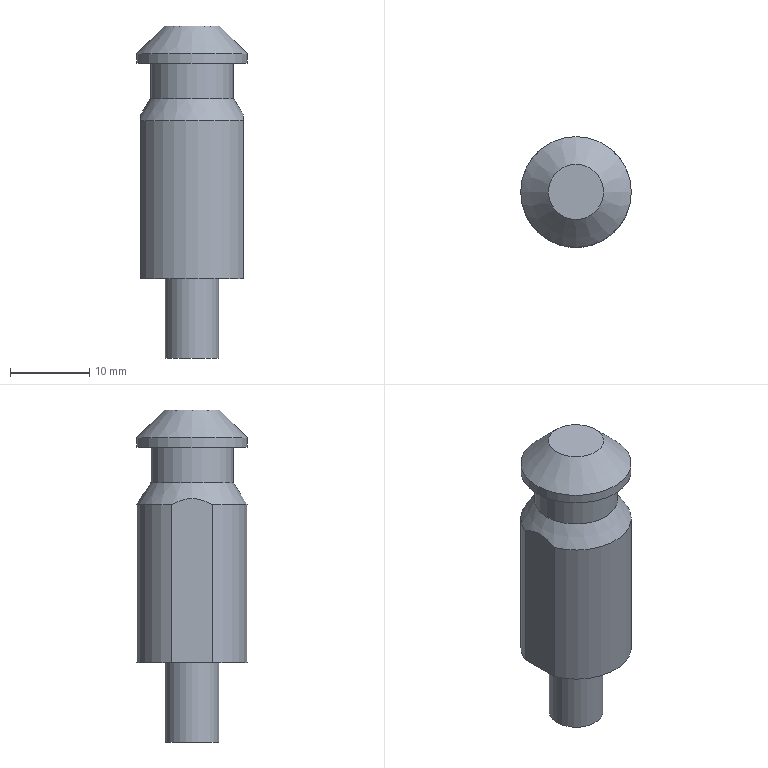Component | NX | PART | 1 solid | 13 faces | box 14 x 14 x 42 mm | volume 4592 mm3 | plane 6 | cylinder 5 | cone 2 | commonest cylinder face diameters 14 x3 6.8 x1 10.501 x1
STEP:
#1=CARTESIAN_POINT('',(0.,0.,0.));
#2=DIRECTION('',(0.,0.,1.));
#3=DIRECTION('',(1.,0.,0.));
#4=AXIS2_PLACEMENT_3D('',#1,#2,#3);
#5=CARTESIAN_POINT('',(-5.25,0.,31.8));
#6=VERTEX_POINT('',#5);
#7=CARTESIAN_POINT('',(-0.,0.,31.8));
#8=DIRECTION('',(0.,0.,-1.));
#9=DIRECTION('',(-1.,0.,0.));
#10=AXIS2_PLACEMENT_3D('',#7,#8,#9);
#11=CIRCLE('',#10,5.25);
#12=CARTESIAN_POINT('',(-0.,0.,31.8));
#13=DIRECTION('',(0.,0.,-1.));
#14=DIRECTION('',(-1.,0.,0.));
#15=AXIS2_PLACEMENT_3D('',#12,#13,#14);
#16=CONICAL_SURFACE('',#15,5.25,0.5585);
#17=CARTESIAN_POINT('',(0.,0.));
#18=DIRECTION('',(1.,0.));
#19=VECTOR('',#18,1.);
#20=LINE('',#17,#19);
#21=(GEOMETRIC_REPRESENTATION_CONTEXT(2)PARAMETRIC_REPRESENTATION_CONTEXT()REPRESENTATION_CONTEXT('',''));
#22=DEFINITIONAL_REPRESENTATION('',(#20),#21);
#23=PCURVE('',#16,#22);
#24=CARTESIAN_POINT('',(-0.,0.,9.));
#25=DIRECTION('',(0.,0.,-1.));
#26=DIRECTION('',(-1.,0.,0.));
#27=AXIS2_PLACEMENT_3D('',#24,#25,#26);
#28=CYLINDRICAL_SURFACE('',#27,5.25);
#29=CARTESIAN_POINT('',(0.,-22.8));
#30=DIRECTION('',(1.,0.));
#31=VECTOR('',#30,1.);
#32=LINE('',#29,#31);
#33=(GEOMETRIC_REPRESENTATION_CONTEXT(2)PARAMETRIC_REPRESENTATION_CONTEXT()REPRESENTATION_CONTEXT('',''));
#34=DEFINITIONAL_REPRESENTATION('',(#32),#33);
#35=PCURVE('',#28,#34);
#36=SURFACE_CURVE('',#11,(#23,#35),.PCURVE_S1.);
#37=EDGE_CURVE('',#6,#6,#36,.T.);
#38=ORIENTED_EDGE('',*,*,#37,.T.);
#39=CARTESIAN_POINT('',(-6.5,0.,29.8));
#40=VERTEX_POINT('',#39);
#41=CARTESIAN_POINT('',(-5.25,0.,31.8));
#42=CARTESIAN_POINT('',(-6.5,0.,29.8));
#43=B_SPLINE_CURVE_WITH_KNOTS('',1,(#41,#42),.UNSPECIFIED.,.F.,.F.,(2,2),(0.,2.358),.PIECEWISE_BEZIER_KNOTS.);
#44=CARTESIAN_POINT('',(6.283,0.));
#45=DIRECTION('',(0.,1.));
#46=VECTOR('',#45,1.);
#47=LINE('',#44,#46);
#48=(GEOMETRIC_REPRESENTATION_CONTEXT(2)PARAMETRIC_REPRESENTATION_CONTEXT()REPRESENTATION_CONTEXT('',''));
#49=DEFINITIONAL_REPRESENTATION('',(#47),#48);
#50=PCURVE('',#16,#49);
#51=CARTESIAN_POINT('',(0.,0.));
#52=DIRECTION('',(0.,1.));
#53=VECTOR('',#52,1.);
#54=LINE('',#51,#53);
#55=(GEOMETRIC_REPRESENTATION_CONTEXT(2)PARAMETRIC_REPRESENTATION_CONTEXT()REPRESENTATION_CONTEXT('',''));
#56=DEFINITIONAL_REPRESENTATION('',(#54),#55);
#57=PCURVE('',#16,#56);
#58=SEAM_CURVE('',#43,(#50,#57),.PCURVE_S1.);
#59=EDGE_CURVE('',#6,#40,#58,.T.);
#60=ORIENTED_EDGE('',*,*,#59,.T.);
#61=CARTESIAN_POINT('',(-6.5,-2.598,29.));
#62=VERTEX_POINT('',#61);
#63=CARTESIAN_POINT('',(-6.5,2.598,29.));
#64=CARTESIAN_POINT('',(-6.5,1.811,29.468));
#65=CARTESIAN_POINT('',(-6.5,0.9224,29.799));
#66=CARTESIAN_POINT('',(-6.5,-0.9091,29.802));
#67=CARTESIAN_POINT('',(-6.5,-1.805,29.471));
#68=CARTESIAN_POINT('',(-6.5,-2.598,29.));
#69=B_SPLINE_CURVE_WITH_KNOTS('',3,(#63,#64,#65,#66,#67,#68),.UNSPECIFIED.,.F.,.F.,(4,2,4),(0.,0.5,1.),.UNSPECIFIED.);
#70=CARTESIAN_POINT('',(6.663,2.8));
#71=CARTESIAN_POINT('',(6.654,2.757));
#72=CARTESIAN_POINT('',(6.635,2.675));
#73=CARTESIAN_POINT('',(6.604,2.558));
#74=CARTESIAN_POINT('',(6.572,2.45));
#75=CARTESIAN_POINT('',(6.54,2.351));
#76=CARTESIAN_POINT('',(6.506,2.262));
#77=CARTESIAN_POINT('',(6.471,2.185));
#78=CARTESIAN_POINT('',(6.435,2.12));
#79=CARTESIAN_POINT('',(6.398,2.068));
#80=CARTESIAN_POINT('',(6.361,2.029));
#81=CARTESIAN_POINT('',(6.323,2.006));
#82=CARTESIAN_POINT('',(6.284,1.997));
#83=CARTESIAN_POINT('',(6.246,2.005));
#84=CARTESIAN_POINT('',(6.208,2.028));
#85=CARTESIAN_POINT('',(6.17,2.066));
#86=CARTESIAN_POINT('',(6.133,2.118));
#87=CARTESIAN_POINT('',(6.097,2.183));
#88=CARTESIAN_POINT('',(6.062,2.26));
#89=CARTESIAN_POINT('',(6.028,2.349));
#90=CARTESIAN_POINT('',(5.995,2.448));
#91=CARTESIAN_POINT('',(5.963,2.556));
#92=CARTESIAN_POINT('',(5.932,2.674));
#93=CARTESIAN_POINT('',(5.912,2.757));
#94=CARTESIAN_POINT('',(5.903,2.8));
#95=B_SPLINE_CURVE_WITH_KNOTS('',3,(#70,#71,#72,#73,#74,#75,#76,#77,#78,#79,#80,#81,#82,#83,#84,#85,#86,#87,#88,#89,#90,#91,#92,#93,#94),.UNSPECIFIED.,.F.,.F.,(4,1,1,1,1,1,1,1,1,1,1,1,1,1,1,1,1,1,1,1,1,1,4),(0.,0.04545,0.09091,0.1364,0.1818,0.2273,0.2727,0.3182,0.3636,0.4091,0.4545,0.5,0.5455,0.5909,0.6364,0.6818,0.7273,0.7727,0.8182,0.8636,0.9091,0.9545,1.),.QUASI_UNIFORM_KNOTS.);
#96=(GEOMETRIC_REPRESENTATION_CONTEXT(2)PARAMETRIC_REPRESENTATION_CONTEXT()REPRESENTATION_CONTEXT('',''));
#97=DEFINITIONAL_REPRESENTATION('',(#95),#96);
#98=PCURVE('',#16,#97);
#99=CARTESIAN_POINT('',(-6.5,-6.7,35.5));
#100=DIRECTION('',(-1.,0.,0.));
#101=DIRECTION('',(0.,0.,1.));
#102=AXIS2_PLACEMENT_3D('',#99,#100,#101);
#103=PLANE('',#102);
#104=CARTESIAN_POINT('',(-6.5,9.298));
#105=CARTESIAN_POINT('',(-6.032,8.511));
#106=CARTESIAN_POINT('',(-5.701,7.622));
#107=CARTESIAN_POINT('',(-5.698,5.791));
#108=CARTESIAN_POINT('',(-6.029,4.895));
#109=CARTESIAN_POINT('',(-6.5,4.102));
#110=B_SPLINE_CURVE_WITH_KNOTS('',3,(#104,#105,#106,#107,#108,#109),.UNSPECIFIED.,.F.,.F.,(4,2,4),(0.,0.5,1.),.UNSPECIFIED.);
#111=(GEOMETRIC_REPRESENTATION_CONTEXT(2)PARAMETRIC_REPRESENTATION_CONTEXT()REPRESENTATION_CONTEXT('',''));
#112=DEFINITIONAL_REPRESENTATION('',(#110),#111);
#113=PCURVE('',#103,#112);
#114=SURFACE_CURVE('',#69,(#98,#113),.PCURVE_S1.);
#115=EDGE_CURVE('',#40,#62,#114,.T.);
#116=ORIENTED_EDGE('',*,*,#115,.T.);
#117=CARTESIAN_POINT('',(6.5,-2.598,29.));
#118=VERTEX_POINT('',#117);
#119=CARTESIAN_POINT('',(-0.,0.,29.));
#120=DIRECTION('',(0.,0.,-1.));
#121=DIRECTION('',(1.,0.,0.));
#122=AXIS2_PLACEMENT_3D('',#119,#120,#121);
#123=CIRCLE('',#122,7.);
#124=CARTESIAN_POINT('',(3.142,2.8));
#125=DIRECTION('',(1.,0.));
#126=VECTOR('',#125,1.);
#127=LINE('',#124,#126);
#128=(GEOMETRIC_REPRESENTATION_CONTEXT(2)PARAMETRIC_REPRESENTATION_CONTEXT()REPRESENTATION_CONTEXT('',''));
#129=DEFINITIONAL_REPRESENTATION('',(#127),#128);
#130=PCURVE('',#16,#129);
#131=CARTESIAN_POINT('',(-0.,0.,9.));
#132=DIRECTION('',(0.,0.,1.));
#133=DIRECTION('',(1.,0.,0.));
#134=AXIS2_PLACEMENT_3D('',#131,#132,#133);
#135=CYLINDRICAL_SURFACE('',#134,7.);
#136=CARTESIAN_POINT('',(6.283,20.));
#137=DIRECTION('',(-1.,0.));
#138=VECTOR('',#137,1.);
#139=LINE('',#136,#138);
#140=(GEOMETRIC_REPRESENTATION_CONTEXT(2)PARAMETRIC_REPRESENTATION_CONTEXT()REPRESENTATION_CONTEXT('',''));
#141=DEFINITIONAL_REPRESENTATION('',(#139),#140);
#142=PCURVE('',#135,#141);
#143=SURFACE_CURVE('',#123,(#130,#142),.PCURVE_S1.);
#144=EDGE_CURVE('',#118,#62,#143,.T.);
#145=ORIENTED_EDGE('',*,*,#144,.F.);
#146=CARTESIAN_POINT('',(6.5,2.598,29.));
#147=VERTEX_POINT('',#146);
#148=CARTESIAN_POINT('',(6.5,2.598,29.));
#149=CARTESIAN_POINT('',(6.5,1.811,29.468));
#150=CARTESIAN_POINT('',(6.5,0.9224,29.799));
#151=CARTESIAN_POINT('',(6.5,-0.9091,29.802));
#152=CARTESIAN_POINT('',(6.5,-1.805,29.471));
#153=CARTESIAN_POINT('',(6.5,-2.598,29.));
#154=B_SPLINE_CURVE_WITH_KNOTS('',3,(#148,#149,#150,#151,#152,#153),.UNSPECIFIED.,.F.,.F.,(4,2,4),(0.,0.5,1.),.UNSPECIFIED.);
#155=CARTESIAN_POINT('',(2.761,2.8));
#156=CARTESIAN_POINT('',(2.771,2.757));
#157=CARTESIAN_POINT('',(2.79,2.675));
#158=CARTESIAN_POINT('',(2.821,2.558));
#159=CARTESIAN_POINT('',(2.852,2.45));
#160=CARTESIAN_POINT('',(2.885,2.351));
#161=CARTESIAN_POINT('',(2.919,2.262));
#162=CARTESIAN_POINT('',(2.954,2.185));
#163=CARTESIAN_POINT('',(2.99,2.12));
#164=CARTESIAN_POINT('',(3.027,2.068));
#165=CARTESIAN_POINT('',(3.064,2.029));
#166=CARTESIAN_POINT('',(3.102,2.006));
#167=CARTESIAN_POINT('',(3.141,1.997));
#168=CARTESIAN_POINT('',(3.179,2.005));
#169=CARTESIAN_POINT('',(3.217,2.028));
#170=CARTESIAN_POINT('',(3.255,2.066));
#171=CARTESIAN_POINT('',(3.291,2.118));
#172=CARTESIAN_POINT('',(3.328,2.183));
#173=CARTESIAN_POINT('',(3.363,2.26));
#174=CARTESIAN_POINT('',(3.397,2.349));
#175=CARTESIAN_POINT('',(3.43,2.448));
#176=CARTESIAN_POINT('',(3.462,2.556));
#177=CARTESIAN_POINT('',(3.493,2.674));
#178=CARTESIAN_POINT('',(3.512,2.757));
#179=CARTESIAN_POINT('',(3.522,2.8));
#180=B_SPLINE_CURVE_WITH_KNOTS('',3,(#155,#156,#157,#158,#159,#160,#161,#162,#163,#164,#165,#166,#167,#168,#169,#170,#171,#172,#173,#174,#175,#176,#177,#178,#179),.UNSPECIFIED.,.F.,.F.,(4,1,1,1,1,1,1,1,1,1,1,1,1,1,1,1,1,1,1,1,1,1,4),(0.,0.04545,0.09091,0.1364,0.1818,0.2273,0.2727,0.3182,0.3636,0.4091,0.4545,0.5,0.5455,0.5909,0.6364,0.6818,0.7273,0.7727,0.8182,0.8636,0.9091,0.9545,1.),.QUASI_UNIFORM_KNOTS.);
#181=(GEOMETRIC_REPRESENTATION_CONTEXT(2)PARAMETRIC_REPRESENTATION_CONTEXT()REPRESENTATION_CONTEXT('',''));
#182=DEFINITIONAL_REPRESENTATION('',(#180),#181);
#183=PCURVE('',#16,#182);
#184=CARTESIAN_POINT('',(6.5,-6.7,35.5));
#185=DIRECTION('',(-1.,0.,0.));
#186=DIRECTION('',(0.,0.,1.));
#187=AXIS2_PLACEMENT_3D('',#184,#185,#186);
#188=PLANE('',#187);
#189=CARTESIAN_POINT('',(-6.5,9.298));
#190=CARTESIAN_POINT('',(-6.032,8.511));
#191=CARTESIAN_POINT('',(-5.701,7.622));
#192=CARTESIAN_POINT('',(-5.698,5.791));
#193=CARTESIAN_POINT('',(-6.029,4.895));
#194=CARTESIAN_POINT('',(-6.5,4.102));
#195=B_SPLINE_CURVE_WITH_KNOTS('',3,(#189,#190,#191,#192,#193,#194),.UNSPECIFIED.,.F.,.F.,(4,2,4),(0.,0.5,1.),.UNSPECIFIED.);
#196=(GEOMETRIC_REPRESENTATION_CONTEXT(2)PARAMETRIC_REPRESENTATION_CONTEXT()REPRESENTATION_CONTEXT('',''));
#197=DEFINITIONAL_REPRESENTATION('',(#195),#196);
#198=PCURVE('',#188,#197);
#199=SURFACE_CURVE('',#154,(#183,#198),.PCURVE_S1.);
#200=EDGE_CURVE('',#147,#118,#199,.T.);
#201=ORIENTED_EDGE('',*,*,#200,.F.);
#202=CARTESIAN_POINT('',(-6.5,2.598,29.));
#203=VERTEX_POINT('',#202);
#204=CARTESIAN_POINT('',(-0.,0.,29.));
#205=DIRECTION('',(0.,0.,-1.));
#206=DIRECTION('',(1.,0.,0.));
#207=AXIS2_PLACEMENT_3D('',#204,#205,#206);
#208=CIRCLE('',#207,7.);
#209=CARTESIAN_POINT('',(-3.142,2.8));
#210=DIRECTION('',(1.,0.));
#211=VECTOR('',#210,1.);
#212=LINE('',#209,#211);
#213=(GEOMETRIC_REPRESENTATION_CONTEXT(2)PARAMETRIC_REPRESENTATION_CONTEXT()REPRESENTATION_CONTEXT('',''));
#214=DEFINITIONAL_REPRESENTATION('',(#212),#213);
#215=PCURVE('',#16,#214);
#216=CARTESIAN_POINT('',(-0.,0.,9.));
#217=DIRECTION('',(0.,0.,1.));
#218=DIRECTION('',(1.,0.,0.));
#219=AXIS2_PLACEMENT_3D('',#216,#217,#218);
#220=CYLINDRICAL_SURFACE('',#219,7.);
#221=CARTESIAN_POINT('',(6.283,20.));
#222=DIRECTION('',(-1.,0.));
#223=VECTOR('',#222,1.);
#224=LINE('',#221,#223);
#225=(GEOMETRIC_REPRESENTATION_CONTEXT(2)PARAMETRIC_REPRESENTATION_CONTEXT()REPRESENTATION_CONTEXT('',''));
#226=DEFINITIONAL_REPRESENTATION('',(#224),#225);
#227=PCURVE('',#220,#226);
#228=SURFACE_CURVE('',#208,(#215,#227),.PCURVE_S1.);
#229=EDGE_CURVE('',#203,#147,#228,.T.);
#230=ORIENTED_EDGE('',*,*,#229,.F.);
#231=CARTESIAN_POINT('',(-6.5,2.598,29.));
#232=CARTESIAN_POINT('',(-6.5,1.811,29.468));
#233=CARTESIAN_POINT('',(-6.5,0.9224,29.799));
#234=CARTESIAN_POINT('',(-6.5,-0.9091,29.802));
#235=CARTESIAN_POINT('',(-6.5,-1.805,29.471));
#236=CARTESIAN_POINT('',(-6.5,-2.598,29.));
#237=B_SPLINE_CURVE_WITH_KNOTS('',3,(#231,#232,#233,#234,#235,#236),.UNSPECIFIED.,.F.,.F.,(4,2,4),(0.,0.5,1.),.UNSPECIFIED.);
#238=CARTESIAN_POINT('',(0.3803,2.8));
#239=CARTESIAN_POINT('',(0.3708,2.757));
#240=CARTESIAN_POINT('',(0.3513,2.675));
#241=CARTESIAN_POINT('',(0.3209,2.558));
#242=CARTESIAN_POINT('',(0.2892,2.45));
#243=CARTESIAN_POINT('',(0.2564,2.351));
#244=CARTESIAN_POINT('',(0.2224,2.262));
#245=CARTESIAN_POINT('',(0.1874,2.185));
#246=CARTESIAN_POINT('',(0.1515,2.12));
#247=CARTESIAN_POINT('',(0.1147,2.068));
#248=CARTESIAN_POINT('',(0.07732,2.029));
#249=CARTESIAN_POINT('',(0.03938,2.006));
#250=CARTESIAN_POINT('',(0.001028,1.997));
#251=CARTESIAN_POINT('',(-0.03736,2.005));
#252=CARTESIAN_POINT('',(-0.07538,2.028));
#253=CARTESIAN_POINT('',(-0.1129,2.066));
#254=CARTESIAN_POINT('',(-0.1498,2.118));
#255=CARTESIAN_POINT('',(-0.186,2.183));
#256=CARTESIAN_POINT('',(-0.2212,2.26));
#257=CARTESIAN_POINT('',(-0.2554,2.349));
#258=CARTESIAN_POINT('',(-0.2885,2.448));
#259=CARTESIAN_POINT('',(-0.3205,2.556));
#260=CARTESIAN_POINT('',(-0.3511,2.674));
#261=CARTESIAN_POINT('',(-0.3707,2.757));
#262=CARTESIAN_POINT('',(-0.3803,2.8));
#263=B_SPLINE_CURVE_WITH_KNOTS('',3,(#238,#239,#240,#241,#242,#243,#244,#245,#246,#247,#248,#249,#250,#251,#252,#253,#254,#255,#256,#257,#258,#259,#260,#261,#262),.UNSPECIFIED.,.F.,.F.,(4,1,1,1,1,1,1,1,1,1,1,1,1,1,1,1,1,1,1,1,1,1,4),(0.,0.04545,0.09091,0.1364,0.1818,0.2273,0.2727,0.3182,0.3636,0.4091,0.4545,0.5,0.5455,0.5909,0.6364,0.6818,0.7273,0.7727,0.8182,0.8636,0.9091,0.9545,1.),.QUASI_UNIFORM_KNOTS.);
#264=(GEOMETRIC_REPRESENTATION_CONTEXT(2)PARAMETRIC_REPRESENTATION_CONTEXT()REPRESENTATION_CONTEXT('',''));
#265=DEFINITIONAL_REPRESENTATION('',(#263),#264);
#266=PCURVE('',#16,#265);
#267=CARTESIAN_POINT('',(-6.5,9.298));
#268=CARTESIAN_POINT('',(-6.032,8.511));
#269=CARTESIAN_POINT('',(-5.701,7.622));
#270=CARTESIAN_POINT('',(-5.698,5.791));
#271=CARTESIAN_POINT('',(-6.029,4.895));
#272=CARTESIAN_POINT('',(-6.5,4.102));
#273=B_SPLINE_CURVE_WITH_KNOTS('',3,(#267,#268,#269,#270,#271,#272),.UNSPECIFIED.,.F.,.F.,(4,2,4),(0.,0.5,1.),.UNSPECIFIED.);
#274=(GEOMETRIC_REPRESENTATION_CONTEXT(2)PARAMETRIC_REPRESENTATION_CONTEXT()REPRESENTATION_CONTEXT('',''));
#275=DEFINITIONAL_REPRESENTATION('',(#273),#274);
#276=PCURVE('',#103,#275);
#277=SURFACE_CURVE('',#237,(#266,#276),.PCURVE_S1.);
#278=EDGE_CURVE('',#203,#40,#277,.T.);
#279=ORIENTED_EDGE('',*,*,#278,.T.);
#280=ORIENTED_EDGE('',*,*,#59,.F.);
#281=EDGE_LOOP('',(#38,#60,#116,#145,#201,#230,#279,#280));
#282=FACE_BOUND('',#281,.T.);
#283=ADVANCED_FACE('',(#282),#16,.T.);
#284=CARTESIAN_POINT('',(-3.4,0.,9.));
#285=VERTEX_POINT('',#284);
#286=CARTESIAN_POINT('',(-0.,0.,9.));
#287=DIRECTION('',(0.,0.,-1.));
#288=DIRECTION('',(-1.,0.,0.));
#289=AXIS2_PLACEMENT_3D('',#286,#287,#288);
#290=CIRCLE('',#289,3.4);
#291=CARTESIAN_POINT('',(-0.,0.,9.));
#292=DIRECTION('',(0.,0.,-1.));
#293=DIRECTION('',(-1.,0.,0.));
#294=AXIS2_PLACEMENT_3D('',#291,#292,#293);
#295=PLANE('',#294);
#296=CARTESIAN_POINT('',(0.,0.));
#297=DIRECTION('',(1.,0.));
#298=AXIS2_PLACEMENT_2D('',#296,#297);
#299=CIRCLE('',#298,3.4);
#300=(GEOMETRIC_REPRESENTATION_CONTEXT(2)PARAMETRIC_REPRESENTATION_CONTEXT()REPRESENTATION_CONTEXT('',''));
#301=DEFINITIONAL_REPRESENTATION('',(#299),#300);
#302=PCURVE('',#295,#301);
#303=CARTESIAN_POINT('',(-0.,0.,9.));
#304=DIRECTION('',(0.,0.,-1.));
#305=DIRECTION('',(-1.,0.,0.));
#306=AXIS2_PLACEMENT_3D('',#303,#304,#305);
#307=CYLINDRICAL_SURFACE('',#306,3.4);
#308=CARTESIAN_POINT('',(0.,0.));
#309=DIRECTION('',(1.,0.));
#310=VECTOR('',#309,1.);
#311=LINE('',#308,#310);
#312=(GEOMETRIC_REPRESENTATION_CONTEXT(2)PARAMETRIC_REPRESENTATION_CONTEXT()REPRESENTATION_CONTEXT('',''));
#313=DEFINITIONAL_REPRESENTATION('',(#311),#312);
#314=PCURVE('',#307,#313);
#315=SURFACE_CURVE('',#290,(#302,#314),.PCURVE_S1.);
#316=EDGE_CURVE('',#285,#285,#315,.T.);
#317=ORIENTED_EDGE('',*,*,#316,.F.);
#318=EDGE_LOOP('',(#317));
#319=FACE_BOUND('',#318,.T.);
#320=CARTESIAN_POINT('',(-6.5,-2.598,9.));
#321=VERTEX_POINT('',#320);
#322=CARTESIAN_POINT('',(6.5,-2.598,9.));
#323=VERTEX_POINT('',#322);
#324=CARTESIAN_POINT('',(-0.,0.,9.));
#325=DIRECTION('',(0.,0.,1.));
#326=DIRECTION('',(1.,0.,0.));
#327=AXIS2_PLACEMENT_3D('',#324,#325,#326);
#328=CIRCLE('',#327,7.);
#329=CARTESIAN_POINT('',(-7.,0.));
#330=CARTESIAN_POINT('',(-7.,12.124));
#331=CARTESIAN_POINT('',(3.5,6.062));
#332=CARTESIAN_POINT('',(14.,0.));
#333=CARTESIAN_POINT('',(3.5,-6.062));
#334=CARTESIAN_POINT('',(-7.,-12.124));
#335=CARTESIAN_POINT('',(-7.,0.));
#336=(BOUNDED_CURVE()B_SPLINE_CURVE(2,(#329,#330,#331,#332,#333,#334,#335),.UNSPECIFIED.,.T.,.F.)B_SPLINE_CURVE_WITH_KNOTS((1,2,2,2,2,1),(-2.094,0.,2.094,4.189,6.283,8.378),.UNSPECIFIED.)CURVE()GEOMETRIC_REPRESENTATION_ITEM()RATIONAL_B_SPLINE_CURVE((1.,0.5,1.,0.5,1.,0.5,1.))REPRESENTATION_ITEM(''));
#337=(GEOMETRIC_REPRESENTATION_CONTEXT(2)PARAMETRIC_REPRESENTATION_CONTEXT()REPRESENTATION_CONTEXT('',''));
#338=DEFINITIONAL_REPRESENTATION('',(#336),#337);
#339=PCURVE('',#295,#338);
#340=CARTESIAN_POINT('',(0.,0.));
#341=DIRECTION('',(1.,0.));
#342=VECTOR('',#341,1.);
#343=LINE('',#340,#342);
#344=(GEOMETRIC_REPRESENTATION_CONTEXT(2)PARAMETRIC_REPRESENTATION_CONTEXT()REPRESENTATION_CONTEXT('',''));
#345=DEFINITIONAL_REPRESENTATION('',(#343),#344);
#346=PCURVE('',#135,#345);
#347=SURFACE_CURVE('',#328,(#339,#346),.PCURVE_S1.);
#348=EDGE_CURVE('',#321,#323,#347,.T.);
#349=ORIENTED_EDGE('',*,*,#348,.F.);
#350=CARTESIAN_POINT('',(-6.5,2.598,9.));
#351=VERTEX_POINT('',#350);
#352=CARTESIAN_POINT('',(-6.5,-6.7,9.));
#353=DIRECTION('',(0.,1.,0.));
#354=VECTOR('',#353,1.);
#355=LINE('',#352,#354);
#356=CARTESIAN_POINT('',(6.5,-6.7));
#357=DIRECTION('',(0.,1.));
#358=VECTOR('',#357,1.);
#359=LINE('',#356,#358);
#360=(GEOMETRIC_REPRESENTATION_CONTEXT(2)PARAMETRIC_REPRESENTATION_CONTEXT()REPRESENTATION_CONTEXT('',''));
#361=DEFINITIONAL_REPRESENTATION('',(#359),#360);
#362=PCURVE('',#295,#361);
#363=CARTESIAN_POINT('',(-26.5,0.));
#364=DIRECTION('',(0.,1.));
#365=VECTOR('',#364,1.);
#366=LINE('',#363,#365);
#367=(GEOMETRIC_REPRESENTATION_CONTEXT(2)PARAMETRIC_REPRESENTATION_CONTEXT()REPRESENTATION_CONTEXT('',''));
#368=DEFINITIONAL_REPRESENTATION('',(#366),#367);
#369=PCURVE('',#103,#368);
#370=SURFACE_CURVE('',#355,(#362,#369),.PCURVE_S1.);
#371=EDGE_CURVE('',#321,#351,#370,.T.);
#372=ORIENTED_EDGE('',*,*,#371,.T.);
#373=CARTESIAN_POINT('',(6.5,2.598,9.));
#374=VERTEX_POINT('',#373);
#375=CARTESIAN_POINT('',(-0.,0.,9.));
#376=DIRECTION('',(0.,0.,1.));
#377=DIRECTION('',(1.,0.,0.));
#378=AXIS2_PLACEMENT_3D('',#375,#376,#377);
#379=CIRCLE('',#378,7.);
#380=CARTESIAN_POINT('',(-7.,0.));
#381=CARTESIAN_POINT('',(-7.,12.124));
#382=CARTESIAN_POINT('',(3.5,6.062));
#383=CARTESIAN_POINT('',(14.,0.));
#384=CARTESIAN_POINT('',(3.5,-6.062));
#385=CARTESIAN_POINT('',(-7.,-12.124));
#386=CARTESIAN_POINT('',(-7.,0.));
#387=(BOUNDED_CURVE()B_SPLINE_CURVE(2,(#380,#381,#382,#383,#384,#385,#386),.UNSPECIFIED.,.T.,.F.)B_SPLINE_CURVE_WITH_KNOTS((1,2,2,2,2,1),(-2.094,0.,2.094,4.189,6.283,8.378),.UNSPECIFIED.)CURVE()GEOMETRIC_REPRESENTATION_ITEM()RATIONAL_B_SPLINE_CURVE((1.,0.5,1.,0.5,1.,0.5,1.))REPRESENTATION_ITEM(''));
#388=(GEOMETRIC_REPRESENTATION_CONTEXT(2)PARAMETRIC_REPRESENTATION_CONTEXT()REPRESENTATION_CONTEXT('',''));
#389=DEFINITIONAL_REPRESENTATION('',(#387),#388);
#390=PCURVE('',#295,#389);
#391=CARTESIAN_POINT('',(0.,0.));
#392=DIRECTION('',(1.,0.));
#393=VECTOR('',#392,1.);
#394=LINE('',#391,#393);
#395=(GEOMETRIC_REPRESENTATION_CONTEXT(2)PARAMETRIC_REPRESENTATION_CONTEXT()REPRESENTATION_CONTEXT('',''));
#396=DEFINITIONAL_REPRESENTATION('',(#394),#395);
#397=PCURVE('',#220,#396);
#398=SURFACE_CURVE('',#379,(#390,#397),.PCURVE_S1.);
#399=EDGE_CURVE('',#374,#351,#398,.T.);
#400=ORIENTED_EDGE('',*,*,#399,.F.);
#401=CARTESIAN_POINT('',(6.5,-6.7,9.));
#402=DIRECTION('',(0.,1.,0.));
#403=VECTOR('',#402,1.);
#404=LINE('',#401,#403);
#405=CARTESIAN_POINT('',(-6.5,-6.7));
#406=DIRECTION('',(0.,1.));
#407=VECTOR('',#406,1.);
#408=LINE('',#405,#407);
#409=(GEOMETRIC_REPRESENTATION_CONTEXT(2)PARAMETRIC_REPRESENTATION_CONTEXT()REPRESENTATION_CONTEXT('',''));
#410=DEFINITIONAL_REPRESENTATION('',(#408),#409);
#411=PCURVE('',#295,#410);
#412=CARTESIAN_POINT('',(-26.5,0.));
#413=DIRECTION('',(0.,1.));
#414=VECTOR('',#413,1.);
#415=LINE('',#412,#414);
#416=(GEOMETRIC_REPRESENTATION_CONTEXT(2)PARAMETRIC_REPRESENTATION_CONTEXT()REPRESENTATION_CONTEXT('',''));
#417=DEFINITIONAL_REPRESENTATION('',(#415),#416);
#418=PCURVE('',#188,#417);
#419=SURFACE_CURVE('',#404,(#411,#418),.PCURVE_S1.);
#420=EDGE_CURVE('',#323,#374,#419,.T.);
#421=ORIENTED_EDGE('',*,*,#420,.F.);
#422=EDGE_LOOP('',(#349,#372,#400,#421));
#423=FACE_BOUND('',#422,.T.);
#424=ADVANCED_FACE('',(#319,#423),#295,.T.);
#425=ORIENTED_EDGE('',*,*,#144,.T.);
#426=CARTESIAN_POINT('',(-6.5,-2.598,9.));
#427=DIRECTION('',(0.,0.,-1.));
#428=VECTOR('',#427,1.);
#429=LINE('',#426,#428);
#430=CARTESIAN_POINT('',(3.522,0.));
#431=DIRECTION('',(0.,-1.));
#432=VECTOR('',#431,1.);
#433=LINE('',#430,#432);
#434=(GEOMETRIC_REPRESENTATION_CONTEXT(2)PARAMETRIC_REPRESENTATION_CONTEXT()REPRESENTATION_CONTEXT('',''));
#435=DEFINITIONAL_REPRESENTATION('',(#433),#434);
#436=PCURVE('',#135,#435);
#437=CARTESIAN_POINT('',(-26.5,4.102));
#438=DIRECTION('',(-1.,0.));
#439=VECTOR('',#438,1.);
#440=LINE('',#437,#439);
#441=(GEOMETRIC_REPRESENTATION_CONTEXT(2)PARAMETRIC_REPRESENTATION_CONTEXT()REPRESENTATION_CONTEXT('',''));
#442=DEFINITIONAL_REPRESENTATION('',(#440),#441);
#443=PCURVE('',#103,#442);
#444=SURFACE_CURVE('',#429,(#436,#443),.PCURVE_S1.);
#445=EDGE_CURVE('',#62,#321,#444,.T.);
#446=ORIENTED_EDGE('',*,*,#445,.T.);
#447=ORIENTED_EDGE('',*,*,#348,.T.);
#448=CARTESIAN_POINT('',(6.5,-2.598,9.));
#449=DIRECTION('',(0.,0.,-1.));
#450=VECTOR('',#449,1.);
#451=LINE('',#448,#450);
#452=CARTESIAN_POINT('',(5.903,0.));
#453=DIRECTION('',(0.,-1.));
#454=VECTOR('',#453,1.);
#455=LINE('',#452,#454);
#456=(GEOMETRIC_REPRESENTATION_CONTEXT(2)PARAMETRIC_REPRESENTATION_CONTEXT()REPRESENTATION_CONTEXT('',''));
#457=DEFINITIONAL_REPRESENTATION('',(#455),#456);
#458=PCURVE('',#135,#457);
#459=CARTESIAN_POINT('',(-26.5,4.102));
#460=DIRECTION('',(-1.,0.));
#461=VECTOR('',#460,1.);
#462=LINE('',#459,#461);
#463=(GEOMETRIC_REPRESENTATION_CONTEXT(2)PARAMETRIC_REPRESENTATION_CONTEXT()REPRESENTATION_CONTEXT('',''));
#464=DEFINITIONAL_REPRESENTATION('',(#462),#463);
#465=PCURVE('',#188,#464);
#466=SURFACE_CURVE('',#451,(#458,#465),.PCURVE_S1.);
#467=EDGE_CURVE('',#118,#323,#466,.T.);
#468=ORIENTED_EDGE('',*,*,#467,.F.);
#469=EDGE_LOOP('',(#425,#446,#447,#468));
#470=FACE_BOUND('',#469,.T.);
#471=ADVANCED_FACE('',(#470),#135,.T.);
#472=ORIENTED_EDGE('',*,*,#399,.T.);
#473=CARTESIAN_POINT('',(-6.5,2.598,9.));
#474=DIRECTION('',(0.,0.,1.));
#475=VECTOR('',#474,1.);
#476=LINE('',#473,#475);
#477=CARTESIAN_POINT('',(2.761,0.));
#478=DIRECTION('',(0.,1.));
#479=VECTOR('',#478,1.);
#480=LINE('',#477,#479);
#481=(GEOMETRIC_REPRESENTATION_CONTEXT(2)PARAMETRIC_REPRESENTATION_CONTEXT()REPRESENTATION_CONTEXT('',''));
#482=DEFINITIONAL_REPRESENTATION('',(#480),#481);
#483=PCURVE('',#220,#482);
#484=CARTESIAN_POINT('',(-26.5,9.298));
#485=DIRECTION('',(1.,0.));
#486=VECTOR('',#485,1.);
#487=LINE('',#484,#486);
#488=(GEOMETRIC_REPRESENTATION_CONTEXT(2)PARAMETRIC_REPRESENTATION_CONTEXT()REPRESENTATION_CONTEXT('',''));
#489=DEFINITIONAL_REPRESENTATION('',(#487),#488);
#490=PCURVE('',#103,#489);
#491=SURFACE_CURVE('',#476,(#483,#490),.PCURVE_S1.);
#492=EDGE_CURVE('',#351,#203,#491,.T.);
#493=ORIENTED_EDGE('',*,*,#492,.T.);
#494=ORIENTED_EDGE('',*,*,#229,.T.);
#495=CARTESIAN_POINT('',(6.5,2.598,9.));
#496=DIRECTION('',(0.,0.,1.));
#497=VECTOR('',#496,1.);
#498=LINE('',#495,#497);
#499=CARTESIAN_POINT('',(0.3803,0.));
#500=DIRECTION('',(0.,1.));
#501=VECTOR('',#500,1.);
#502=LINE('',#499,#501);
#503=(GEOMETRIC_REPRESENTATION_CONTEXT(2)PARAMETRIC_REPRESENTATION_CONTEXT()REPRESENTATION_CONTEXT('',''));
#504=DEFINITIONAL_REPRESENTATION('',(#502),#503);
#505=PCURVE('',#220,#504);
#506=CARTESIAN_POINT('',(-26.5,9.298));
#507=DIRECTION('',(1.,0.));
#508=VECTOR('',#507,1.);
#509=LINE('',#506,#508);
#510=(GEOMETRIC_REPRESENTATION_CONTEXT(2)PARAMETRIC_REPRESENTATION_CONTEXT()REPRESENTATION_CONTEXT('',''));
#511=DEFINITIONAL_REPRESENTATION('',(#509),#510);
#512=PCURVE('',#188,#511);
#513=SURFACE_CURVE('',#498,(#505,#512),.PCURVE_S1.);
#514=EDGE_CURVE('',#374,#147,#513,.T.);
#515=ORIENTED_EDGE('',*,*,#514,.F.);
#516=EDGE_LOOP('',(#472,#493,#494,#515));
#517=FACE_BOUND('',#516,.T.);
#518=ADVANCED_FACE('',(#517),#220,.T.);
#519=ORIENTED_EDGE('',*,*,#467,.T.);
#520=ORIENTED_EDGE('',*,*,#420,.T.);
#521=ORIENTED_EDGE('',*,*,#514,.T.);
#522=ORIENTED_EDGE('',*,*,#200,.T.);
#523=EDGE_LOOP('',(#519,#520,#521,#522));
#524=FACE_BOUND('',#523,.T.);
#525=ADVANCED_FACE('',(#524),#188,.F.);
#526=ORIENTED_EDGE('',*,*,#445,.F.);
#527=ORIENTED_EDGE('',*,*,#115,.F.);
#528=ORIENTED_EDGE('',*,*,#278,.F.);
#529=ORIENTED_EDGE('',*,*,#492,.F.);
#530=ORIENTED_EDGE('',*,*,#371,.F.);
#531=EDGE_LOOP('',(#526,#527,#528,#529,#530));
#532=FACE_BOUND('',#531,.T.);
#533=ADVANCED_FACE('',(#532),#103,.T.);
#534=CARTESIAN_POINT('',(-3.4,0.,-1.));
#535=VERTEX_POINT('',#534);
#536=CARTESIAN_POINT('',(-0.,0.,-1.));
#537=DIRECTION('',(0.,0.,-1.));
#538=DIRECTION('',(-1.,0.,0.));
#539=AXIS2_PLACEMENT_3D('',#536,#537,#538);
#540=CIRCLE('',#539,3.4);
#541=CARTESIAN_POINT('',(-0.,0.,-1.));
#542=DIRECTION('',(0.,0.,-1.));
#543=DIRECTION('',(-1.,0.,0.));
#544=AXIS2_PLACEMENT_3D('',#541,#542,#543);
#545=PLANE('',#544);
#546=CARTESIAN_POINT('',(0.,0.));
#547=DIRECTION('',(1.,0.));
#548=AXIS2_PLACEMENT_2D('',#546,#547);
#549=CIRCLE('',#548,3.4);
#550=(GEOMETRIC_REPRESENTATION_CONTEXT(2)PARAMETRIC_REPRESENTATION_CONTEXT()REPRESENTATION_CONTEXT('',''));
#551=DEFINITIONAL_REPRESENTATION('',(#549),#550);
#552=PCURVE('',#545,#551);
#553=CARTESIAN_POINT('',(0.,10.));
#554=DIRECTION('',(1.,0.));
#555=VECTOR('',#554,1.);
#556=LINE('',#553,#555);
#557=(GEOMETRIC_REPRESENTATION_CONTEXT(2)PARAMETRIC_REPRESENTATION_CONTEXT()REPRESENTATION_CONTEXT('',''));
#558=DEFINITIONAL_REPRESENTATION('',(#556),#557);
#559=PCURVE('',#307,#558);
#560=SURFACE_CURVE('',#540,(#552,#559),.PCURVE_S1.);
#561=EDGE_CURVE('',#535,#535,#560,.T.);
#562=ORIENTED_EDGE('',*,*,#561,.T.);
#563=EDGE_LOOP('',(#562));
#564=FACE_BOUND('',#563,.T.);
#565=ADVANCED_FACE('',(#564),#545,.T.);
#566=ORIENTED_EDGE('',*,*,#561,.F.);
#567=CARTESIAN_POINT('',(-3.4,-0.,9.));
#568=CARTESIAN_POINT('',(-3.4,-0.,-1.));
#569=B_SPLINE_CURVE_WITH_KNOTS('',1,(#567,#568),.UNSPECIFIED.,.F.,.F.,(2,2),(0.,10.),.PIECEWISE_BEZIER_KNOTS.);
#570=CARTESIAN_POINT('',(0.,0.));
#571=DIRECTION('',(0.,1.));
#572=VECTOR('',#571,1.);
#573=LINE('',#570,#572);
#574=(GEOMETRIC_REPRESENTATION_CONTEXT(2)PARAMETRIC_REPRESENTATION_CONTEXT()REPRESENTATION_CONTEXT('',''));
#575=DEFINITIONAL_REPRESENTATION('',(#573),#574);
#576=PCURVE('',#307,#575);
#577=CARTESIAN_POINT('',(6.283,0.));
#578=DIRECTION('',(0.,1.));
#579=VECTOR('',#578,1.);
#580=LINE('',#577,#579);
#581=(GEOMETRIC_REPRESENTATION_CONTEXT(2)PARAMETRIC_REPRESENTATION_CONTEXT()REPRESENTATION_CONTEXT('',''));
#582=DEFINITIONAL_REPRESENTATION('',(#580),#581);
#583=PCURVE('',#307,#582);
#584=SEAM_CURVE('',#569,(#576,#583),.PCURVE_S1.);
#585=EDGE_CURVE('',#285,#535,#584,.T.);
#586=ORIENTED_EDGE('',*,*,#585,.F.);
#587=ORIENTED_EDGE('',*,*,#316,.T.);
#588=ORIENTED_EDGE('',*,*,#585,.T.);
#589=EDGE_LOOP('',(#566,#586,#587,#588));
#590=FACE_BOUND('',#589,.T.);
#591=ADVANCED_FACE('',(#590),#307,.T.);
#592=CARTESIAN_POINT('',(-3.5,0.,41.));
#593=VERTEX_POINT('',#592);
#594=CARTESIAN_POINT('',(-0.,0.,41.));
#595=DIRECTION('',(0.,0.,-1.));
#596=DIRECTION('',(-1.,0.,0.));
#597=AXIS2_PLACEMENT_3D('',#594,#595,#596);
#598=CIRCLE('',#597,3.5);
#599=CARTESIAN_POINT('',(-0.,-0.,41.));
#600=DIRECTION('',(0.,0.,-1.));
#601=DIRECTION('',(-1.,0.,0.));
#602=AXIS2_PLACEMENT_3D('',#599,#600,#601);
#603=PLANE('',#602);
#604=CARTESIAN_POINT('',(0.,0.));
#605=DIRECTION('',(1.,0.));
#606=AXIS2_PLACEMENT_2D('',#604,#605);
#607=CIRCLE('',#606,3.5);
#608=(GEOMETRIC_REPRESENTATION_CONTEXT(2)PARAMETRIC_REPRESENTATION_CONTEXT()REPRESENTATION_CONTEXT('',''));
#609=DEFINITIONAL_REPRESENTATION('',(#607),#608);
#610=PCURVE('',#603,#609);
#611=CARTESIAN_POINT('',(-0.,0.,41.));
#612=DIRECTION('',(0.,0.,-1.));
#613=DIRECTION('',(-1.,0.,0.));
#614=AXIS2_PLACEMENT_3D('',#611,#612,#613);
#615=CONICAL_SURFACE('',#614,3.5,0.7854);
#616=CARTESIAN_POINT('',(0.,0.));
#617=DIRECTION('',(1.,0.));
#618=VECTOR('',#617,1.);
#619=LINE('',#616,#618);
#620=(GEOMETRIC_REPRESENTATION_CONTEXT(2)PARAMETRIC_REPRESENTATION_CONTEXT()REPRESENTATION_CONTEXT('',''));
#621=DEFINITIONAL_REPRESENTATION('',(#619),#620);
#622=PCURVE('',#615,#621);
#623=SURFACE_CURVE('',#598,(#610,#622),.PCURVE_S1.);
#624=EDGE_CURVE('',#593,#593,#623,.T.);
#625=ORIENTED_EDGE('',*,*,#624,.F.);
#626=EDGE_LOOP('',(#625));
#627=FACE_BOUND('',#626,.T.);
#628=ADVANCED_FACE('',(#627),#603,.F.);
#629=CARTESIAN_POINT('',(-7.,0.,37.5));
#630=VERTEX_POINT('',#629);
#631=CARTESIAN_POINT('',(-0.,0.,37.5));
#632=DIRECTION('',(0.,0.,-1.));
#633=DIRECTION('',(-1.,0.,0.));
#634=AXIS2_PLACEMENT_3D('',#631,#632,#633);
#635=CIRCLE('',#634,7.);
#636=CARTESIAN_POINT('',(0.,3.5));
#637=DIRECTION('',(1.,0.));
#638=VECTOR('',#637,1.);
#639=LINE('',#636,#638);
#640=(GEOMETRIC_REPRESENTATION_CONTEXT(2)PARAMETRIC_REPRESENTATION_CONTEXT()REPRESENTATION_CONTEXT('',''));
#641=DEFINITIONAL_REPRESENTATION('',(#639),#640);
#642=PCURVE('',#615,#641);
#643=CARTESIAN_POINT('',(-0.,0.,9.));
#644=DIRECTION('',(0.,0.,-1.));
#645=DIRECTION('',(-1.,0.,0.));
#646=AXIS2_PLACEMENT_3D('',#643,#644,#645);
#647=CYLINDRICAL_SURFACE('',#646,7.);
#648=CARTESIAN_POINT('',(0.,-28.5));
#649=DIRECTION('',(1.,0.));
#650=VECTOR('',#649,1.);
#651=LINE('',#648,#650);
#652=(GEOMETRIC_REPRESENTATION_CONTEXT(2)PARAMETRIC_REPRESENTATION_CONTEXT()REPRESENTATION_CONTEXT('',''));
#653=DEFINITIONAL_REPRESENTATION('',(#651),#652);
#654=PCURVE('',#647,#653);
#655=SURFACE_CURVE('',#635,(#642,#654),.PCURVE_S1.);
#656=EDGE_CURVE('',#630,#630,#655,.T.);
#657=ORIENTED_EDGE('',*,*,#656,.F.);
#658=CARTESIAN_POINT('',(-3.5,-0.,41.));
#659=CARTESIAN_POINT('',(-7.,-0.,37.5));
#660=B_SPLINE_CURVE_WITH_KNOTS('',1,(#658,#659),.UNSPECIFIED.,.F.,.F.,(2,2),(0.,4.95),.PIECEWISE_BEZIER_KNOTS.);
#661=CARTESIAN_POINT('',(0.,0.));
#662=DIRECTION('',(0.,1.));
#663=VECTOR('',#662,1.);
#664=LINE('',#661,#663);
#665=(GEOMETRIC_REPRESENTATION_CONTEXT(2)PARAMETRIC_REPRESENTATION_CONTEXT()REPRESENTATION_CONTEXT('',''));
#666=DEFINITIONAL_REPRESENTATION('',(#664),#665);
#667=PCURVE('',#615,#666);
#668=CARTESIAN_POINT('',(6.283,0.));
#669=DIRECTION('',(0.,1.));
#670=VECTOR('',#669,1.);
#671=LINE('',#668,#670);
#672=(GEOMETRIC_REPRESENTATION_CONTEXT(2)PARAMETRIC_REPRESENTATION_CONTEXT()REPRESENTATION_CONTEXT('',''));
#673=DEFINITIONAL_REPRESENTATION('',(#671),#672);
#674=PCURVE('',#615,#673);
#675=SEAM_CURVE('',#660,(#667,#674),.PCURVE_S1.);
#676=EDGE_CURVE('',#593,#630,#675,.T.);
#677=ORIENTED_EDGE('',*,*,#676,.F.);
#678=ORIENTED_EDGE('',*,*,#624,.T.);
#679=ORIENTED_EDGE('',*,*,#676,.T.);
#680=EDGE_LOOP('',(#657,#677,#678,#679));
#681=FACE_BOUND('',#680,.T.);
#682=ADVANCED_FACE('',(#681),#615,.T.);
#683=CARTESIAN_POINT('',(-7.,0.,36.3));
#684=VERTEX_POINT('',#683);
#685=CARTESIAN_POINT('',(-0.,0.,36.3));
#686=DIRECTION('',(0.,0.,-1.));
#687=DIRECTION('',(-1.,0.,0.));
#688=AXIS2_PLACEMENT_3D('',#685,#686,#687);
#689=CIRCLE('',#688,7.);
#690=CARTESIAN_POINT('',(0.,-27.3));
#691=DIRECTION('',(1.,0.));
#692=VECTOR('',#691,1.);
#693=LINE('',#690,#692);
#694=(GEOMETRIC_REPRESENTATION_CONTEXT(2)PARAMETRIC_REPRESENTATION_CONTEXT()REPRESENTATION_CONTEXT('',''));
#695=DEFINITIONAL_REPRESENTATION('',(#693),#694);
#696=PCURVE('',#647,#695);
#697=CARTESIAN_POINT('',(-0.,-7.,36.3));
#698=DIRECTION('',(0.,0.,1.));
#699=DIRECTION('',(1.,0.,0.));
#700=AXIS2_PLACEMENT_3D('',#697,#698,#699);
#701=PLANE('',#700);
#702=CARTESIAN_POINT('',(-7.,7.));
#703=CARTESIAN_POINT('',(-7.,19.124));
#704=CARTESIAN_POINT('',(3.5,13.062));
#705=CARTESIAN_POINT('',(14.,7.));
#706=CARTESIAN_POINT('',(3.5,0.9378));
#707=CARTESIAN_POINT('',(-7.,-5.124));
#708=CARTESIAN_POINT('',(-7.,7.));
#709=(BOUNDED_CURVE()B_SPLINE_CURVE(2,(#702,#703,#704,#705,#706,#707,#708),.UNSPECIFIED.,.T.,.F.)B_SPLINE_CURVE_WITH_KNOTS((1,2,2,2,2,1),(-2.094,0.,2.094,4.189,6.283,8.378),.UNSPECIFIED.)CURVE()GEOMETRIC_REPRESENTATION_ITEM()RATIONAL_B_SPLINE_CURVE((1.,0.5,1.,0.5,1.,0.5,1.))REPRESENTATION_ITEM(''));
#710=(GEOMETRIC_REPRESENTATION_CONTEXT(2)PARAMETRIC_REPRESENTATION_CONTEXT()REPRESENTATION_CONTEXT('',''));
#711=DEFINITIONAL_REPRESENTATION('',(#709),#710);
#712=PCURVE('',#701,#711);
#713=SURFACE_CURVE('',#689,(#696,#712),.PCURVE_S1.);
#714=EDGE_CURVE('',#684,#684,#713,.T.);
#715=ORIENTED_EDGE('',*,*,#714,.F.);
#716=CARTESIAN_POINT('',(-7.,-0.,37.5));
#717=CARTESIAN_POINT('',(-7.,-0.,36.3));
#718=B_SPLINE_CURVE_WITH_KNOTS('',1,(#716,#717),.UNSPECIFIED.,.F.,.F.,(2,2),(-28.5,-27.3),.PIECEWISE_BEZIER_KNOTS.);
#719=CARTESIAN_POINT('',(0.,0.));
#720=DIRECTION('',(0.,1.));
#721=VECTOR('',#720,1.);
#722=LINE('',#719,#721);
#723=(GEOMETRIC_REPRESENTATION_CONTEXT(2)PARAMETRIC_REPRESENTATION_CONTEXT()REPRESENTATION_CONTEXT('',''));
#724=DEFINITIONAL_REPRESENTATION('',(#722),#723);
#725=PCURVE('',#647,#724);
#726=CARTESIAN_POINT('',(6.283,0.));
#727=DIRECTION('',(0.,1.));
#728=VECTOR('',#727,1.);
#729=LINE('',#726,#728);
#730=(GEOMETRIC_REPRESENTATION_CONTEXT(2)PARAMETRIC_REPRESENTATION_CONTEXT()REPRESENTATION_CONTEXT('',''));
#731=DEFINITIONAL_REPRESENTATION('',(#729),#730);
#732=PCURVE('',#647,#731);
#733=SEAM_CURVE('',#718,(#725,#732),.PCURVE_S1.);
#734=EDGE_CURVE('',#630,#684,#733,.T.);
#735=ORIENTED_EDGE('',*,*,#734,.F.);
#736=ORIENTED_EDGE('',*,*,#656,.T.);
#737=ORIENTED_EDGE('',*,*,#734,.T.);
#738=EDGE_LOOP('',(#715,#735,#736,#737));
#739=FACE_BOUND('',#738,.T.);
#740=ADVANCED_FACE('',(#739),#647,.T.);
#741=CARTESIAN_POINT('',(-5.25,0.,36.3));
#742=VERTEX_POINT('',#741);
#743=CARTESIAN_POINT('',(-0.,0.,36.3));
#744=DIRECTION('',(0.,0.,-1.));
#745=DIRECTION('',(-1.,0.,0.));
#746=AXIS2_PLACEMENT_3D('',#743,#744,#745);
#747=CIRCLE('',#746,5.25);
#748=CARTESIAN_POINT('',(-5.25,7.));
#749=CARTESIAN_POINT('',(-5.25,16.094));
#750=CARTESIAN_POINT('',(2.625,11.547));
#751=CARTESIAN_POINT('',(10.501,7.));
#752=CARTESIAN_POINT('',(2.625,2.453));
#753=CARTESIAN_POINT('',(-5.25,-2.094));
#754=CARTESIAN_POINT('',(-5.25,7.));
#755=(BOUNDED_CURVE()B_SPLINE_CURVE(2,(#748,#749,#750,#751,#752,#753,#754),.UNSPECIFIED.,.T.,.F.)B_SPLINE_CURVE_WITH_KNOTS((1,2,2,2,2,1),(-2.094,0.,2.094,4.189,6.283,8.378),.UNSPECIFIED.)CURVE()GEOMETRIC_REPRESENTATION_ITEM()RATIONAL_B_SPLINE_CURVE((1.,0.5,1.,0.5,1.,0.5,1.))REPRESENTATION_ITEM(''));
#756=(GEOMETRIC_REPRESENTATION_CONTEXT(2)PARAMETRIC_REPRESENTATION_CONTEXT()REPRESENTATION_CONTEXT('',''));
#757=DEFINITIONAL_REPRESENTATION('',(#755),#756);
#758=PCURVE('',#701,#757);
#759=CARTESIAN_POINT('',(0.,-27.3));
#760=DIRECTION('',(1.,0.));
#761=VECTOR('',#760,1.);
#762=LINE('',#759,#761);
#763=(GEOMETRIC_REPRESENTATION_CONTEXT(2)PARAMETRIC_REPRESENTATION_CONTEXT()REPRESENTATION_CONTEXT('',''));
#764=DEFINITIONAL_REPRESENTATION('',(#762),#763);
#765=PCURVE('',#28,#764);
#766=SURFACE_CURVE('',#747,(#758,#765),.PCURVE_S1.);
#767=EDGE_CURVE('',#742,#742,#766,.T.);
#768=ORIENTED_EDGE('',*,*,#767,.F.);
#769=EDGE_LOOP('',(#768));
#770=FACE_BOUND('',#769,.T.);
#771=ORIENTED_EDGE('',*,*,#714,.T.);
#772=EDGE_LOOP('',(#771));
#773=FACE_BOUND('',#772,.T.);
#774=ADVANCED_FACE('',(#770,#773),#701,.F.);
#775=ORIENTED_EDGE('',*,*,#37,.F.);
#776=CARTESIAN_POINT('',(-5.25,-0.,36.3));
#777=CARTESIAN_POINT('',(-5.25,-0.,31.8));
#778=B_SPLINE_CURVE_WITH_KNOTS('',1,(#776,#777),.UNSPECIFIED.,.F.,.F.,(2,2),(-27.3,-22.8),.PIECEWISE_BEZIER_KNOTS.);
#779=CARTESIAN_POINT('',(0.,0.));
#780=DIRECTION('',(0.,1.));
#781=VECTOR('',#780,1.);
#782=LINE('',#779,#781);
#783=(GEOMETRIC_REPRESENTATION_CONTEXT(2)PARAMETRIC_REPRESENTATION_CONTEXT()REPRESENTATION_CONTEXT('',''));
#784=DEFINITIONAL_REPRESENTATION('',(#782),#783);
#785=PCURVE('',#28,#784);
#786=CARTESIAN_POINT('',(6.283,0.));
#787=DIRECTION('',(0.,1.));
#788=VECTOR('',#787,1.);
#789=LINE('',#786,#788);
#790=(GEOMETRIC_REPRESENTATION_CONTEXT(2)PARAMETRIC_REPRESENTATION_CONTEXT()REPRESENTATION_CONTEXT('',''));
#791=DEFINITIONAL_REPRESENTATION('',(#789),#790);
#792=PCURVE('',#28,#791);
#793=SEAM_CURVE('',#778,(#785,#792),.PCURVE_S1.);
#794=EDGE_CURVE('',#742,#6,#793,.T.);
#795=ORIENTED_EDGE('',*,*,#794,.F.);
#796=ORIENTED_EDGE('',*,*,#767,.T.);
#797=ORIENTED_EDGE('',*,*,#794,.T.);
#798=EDGE_LOOP('',(#775,#795,#796,#797));
#799=FACE_BOUND('',#798,.T.);
#800=ADVANCED_FACE('',(#799),#28,.T.);
#801=CLOSED_SHELL('',(#283,#424,#471,#518,#525,#533,#565,#591,#628,#682,#740,#774,#800));
#802=MANIFOLD_SOLID_BREP('',#801);
#803=(LENGTH_UNIT()NAMED_UNIT(*)SI_UNIT(.MILLI.,.METRE.));
#804=UNCERTAINTY_MEASURE_WITH_UNIT(LENGTH_MEASURE(0.0005),#803,'','');
#805=(NAMED_UNIT(*)PLANE_ANGLE_UNIT()SI_UNIT($,.RADIAN.));
#806=(NAMED_UNIT(*)SI_UNIT($,.STERADIAN.)SOLID_ANGLE_UNIT());
#807=(GEOMETRIC_REPRESENTATION_CONTEXT(3)GLOBAL_UNCERTAINTY_ASSIGNED_CONTEXT((#804))GLOBAL_UNIT_ASSIGNED_CONTEXT((#803,#805,#806))REPRESENTATION_CONTEXT('',''));
#808=ADVANCED_BREP_SHAPE_REPRESENTATION('',(#4,#802),#807);